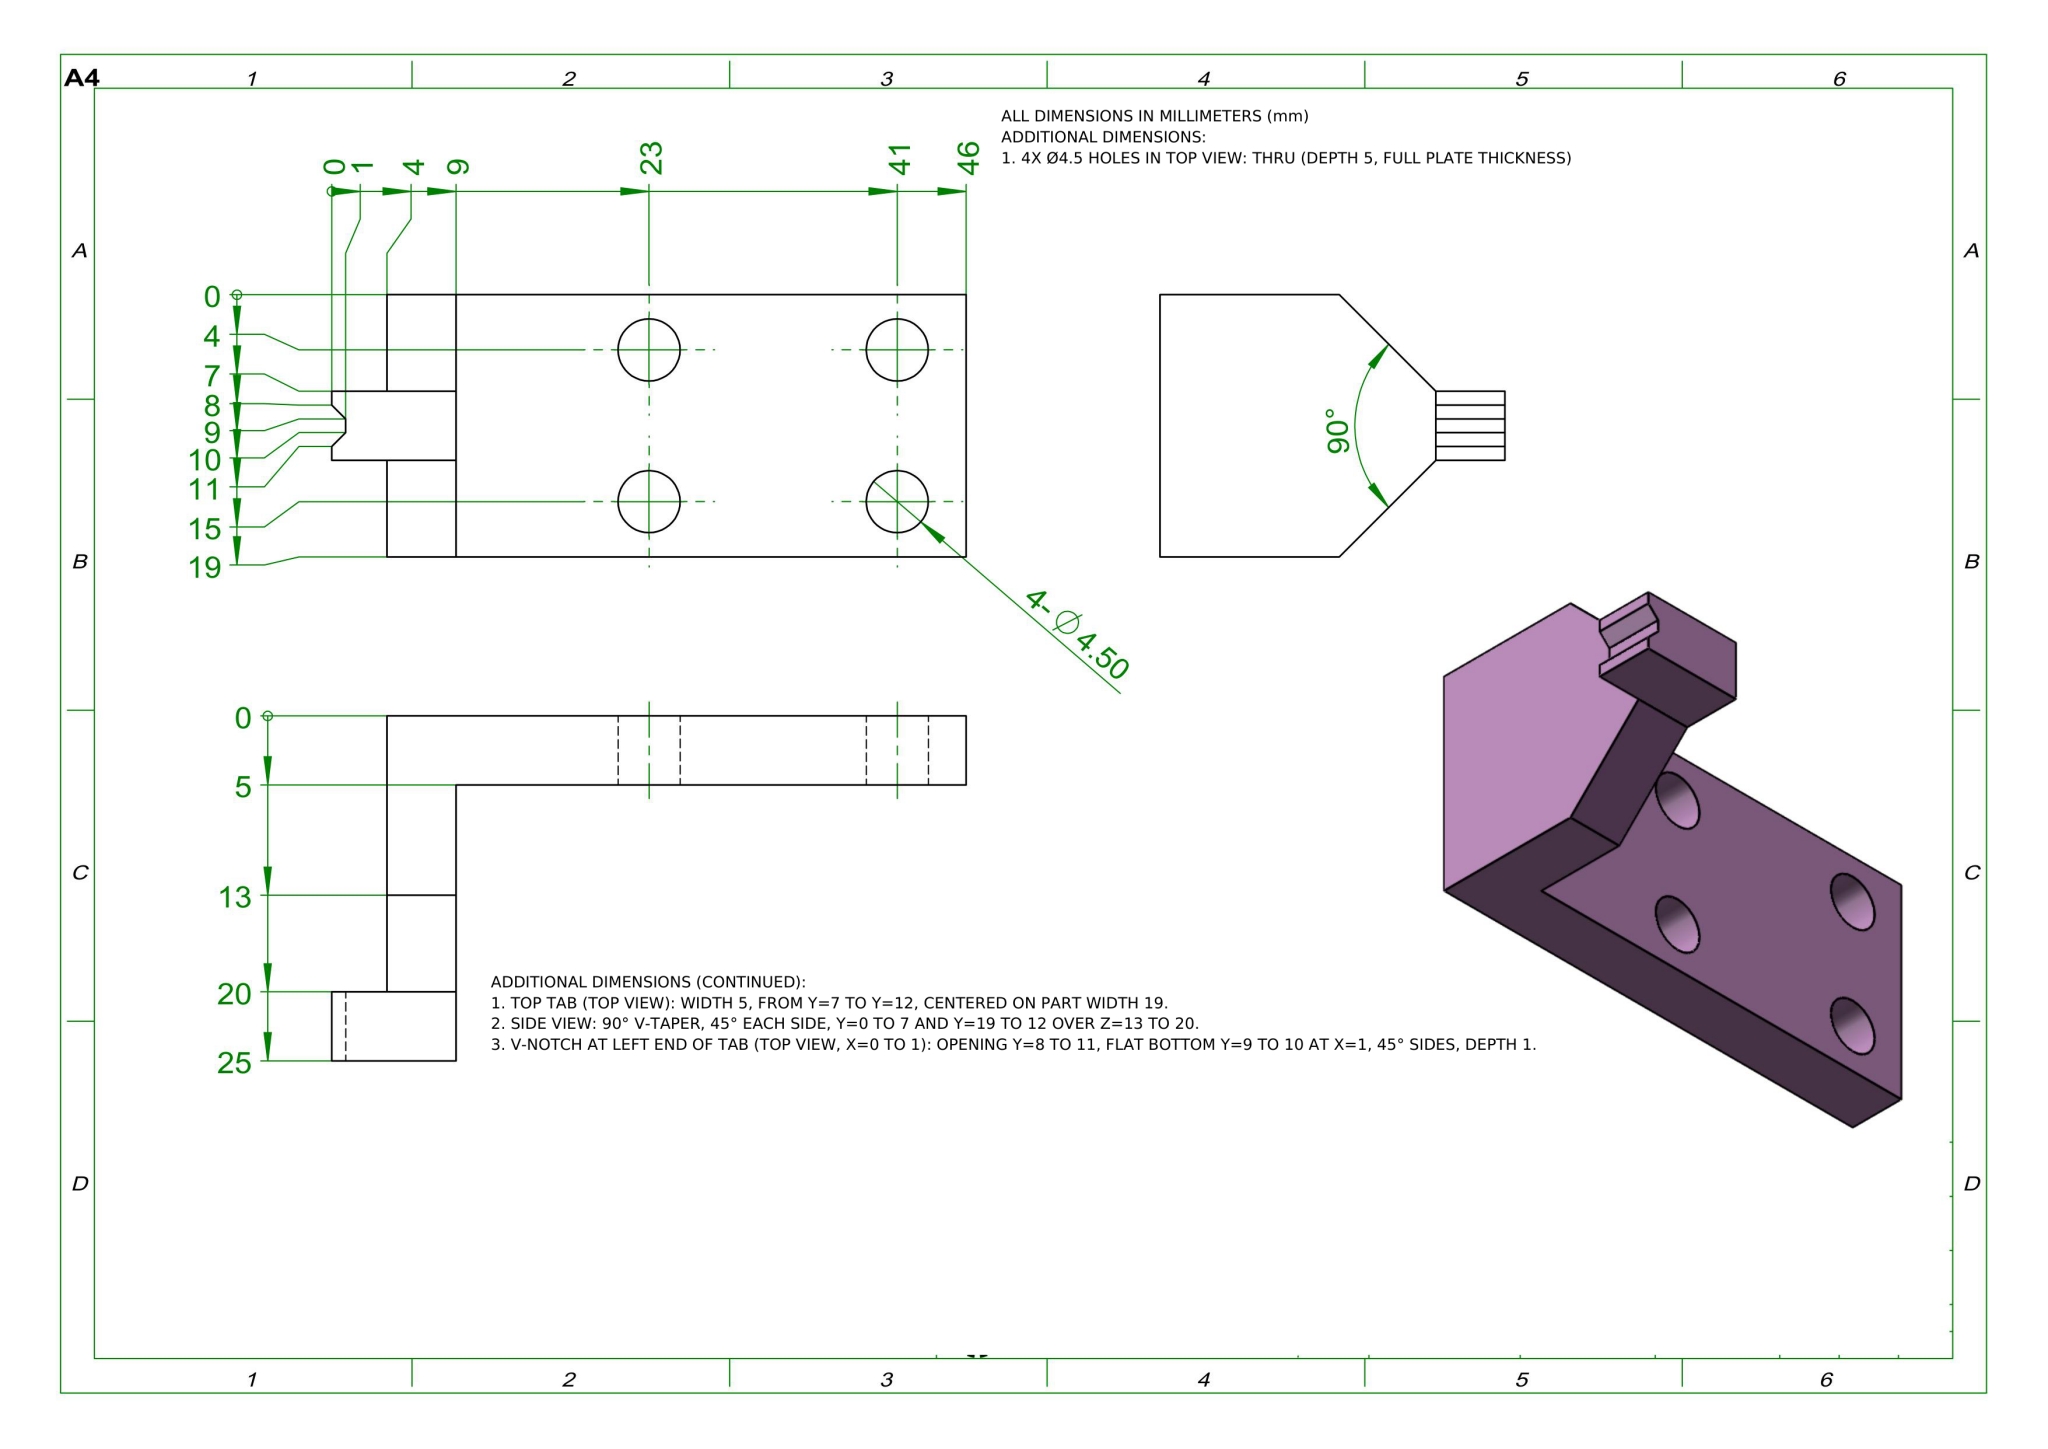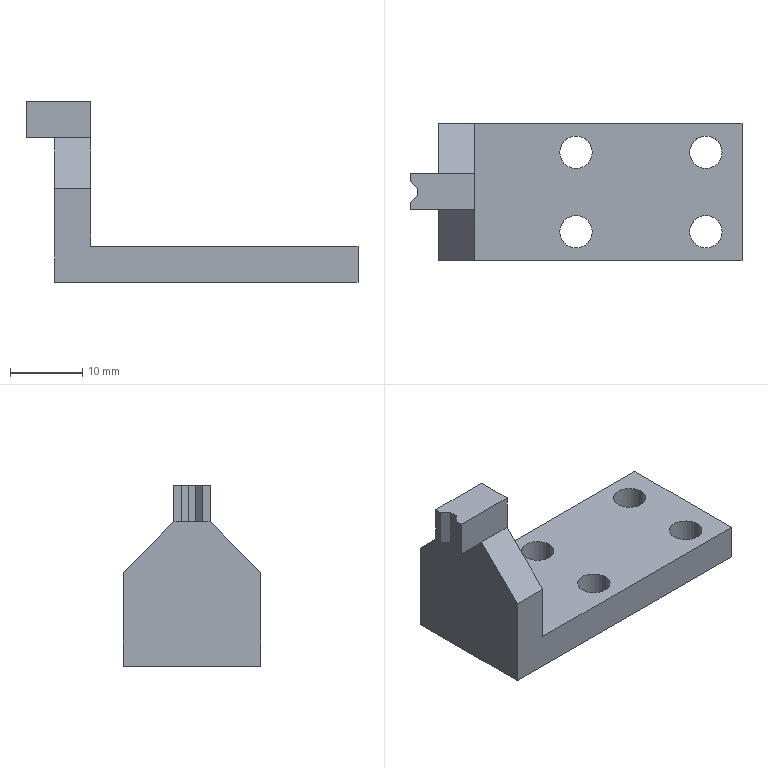Part | NX | mm | 1 solid | 26 faces | box 46 x 19 x 25 mm | volume 5067 mm3 | plane 18 | cylinder 8 | commonest cylinder face diameters 4.5 x8
STEP:
#1=COLOUR_RGB('',1.,0.7529,1.);
#2=FILL_AREA_STYLE_COLOUR('',#1);
#3=FILL_AREA_STYLE('',(#2));
#4=SURFACE_STYLE_FILL_AREA(#3);
#5=SURFACE_SIDE_STYLE('',(#4));
#6=SURFACE_STYLE_USAGE(.BOTH.,#5);
#7=PRESENTATION_STYLE_ASSIGNMENT((#6));
#8=CARTESIAN_POINT('',(-4.25,-5.5,0.));
#9=VERTEX_POINT('',#8);
#10=CARTESIAN_POINT('',(0.25,-5.5,0.));
#11=VERTEX_POINT('',#10);
#12=CARTESIAN_POINT('',(-2.,-5.5,0.));
#13=DIRECTION('',(0.,0.,1.));
#14=DIRECTION('',(-1.,0.,0.));
#15=AXIS2_PLACEMENT_3D('',#12,#13,#14);
#16=CIRCLE('',#15,2.25);
#17=EDGE_CURVE('',#9,#11,#16,.T.);
#18=ORIENTED_EDGE('',*,*,#17,.F.);
#19=CARTESIAN_POINT('',(-4.25,-5.5,5.));
#20=VERTEX_POINT('',#19);
#21=CARTESIAN_POINT('',(-4.25,-5.5,0.));
#22=DIRECTION('',(0.,0.,1.));
#23=VECTOR('',#22,1000.);
#24=LINE('',#21,#23);
#25=EDGE_CURVE('',#9,#20,#24,.T.);
#26=ORIENTED_EDGE('',*,*,#25,.T.);
#27=CARTESIAN_POINT('',(0.25,-5.5,5.));
#28=VERTEX_POINT('',#27);
#29=CARTESIAN_POINT('',(-2.,-5.5,5.));
#30=DIRECTION('',(0.,0.,1.));
#31=DIRECTION('',(-1.,0.,0.));
#32=AXIS2_PLACEMENT_3D('',#29,#30,#31);
#33=CIRCLE('',#32,2.25);
#34=EDGE_CURVE('',#20,#28,#33,.T.);
#35=ORIENTED_EDGE('',*,*,#34,.T.);
#36=CARTESIAN_POINT('',(0.25,-5.5,0.));
#37=DIRECTION('',(0.,0.,1.));
#38=VECTOR('',#37,1000.);
#39=LINE('',#36,#38);
#40=EDGE_CURVE('',#11,#28,#39,.T.);
#41=ORIENTED_EDGE('',*,*,#40,.F.);
#42=EDGE_LOOP('',(#18,#26,#35,#41));
#43=FACE_OUTER_BOUND('',#42,.T.);
#44=CARTESIAN_POINT('',(-2.,-5.5,0.));
#45=DIRECTION('',(0.,0.,1.));
#46=DIRECTION('',(1.,0.,0.));
#47=AXIS2_PLACEMENT_3D('',#44,#45,#46);
#48=CYLINDRICAL_SURFACE('',#47,2.25);
#49=ADVANCED_FACE('',(#43),#48,.F.);
#50=CARTESIAN_POINT('',(13.75,-5.5,0.));
#51=VERTEX_POINT('',#50);
#52=CARTESIAN_POINT('',(18.25,-5.5,0.));
#53=VERTEX_POINT('',#52);
#54=CARTESIAN_POINT('',(16.,-5.5,0.));
#55=DIRECTION('',(0.,0.,1.));
#56=DIRECTION('',(-1.,0.,0.));
#57=AXIS2_PLACEMENT_3D('',#54,#55,#56);
#58=CIRCLE('',#57,2.25);
#59=EDGE_CURVE('',#51,#53,#58,.T.);
#60=ORIENTED_EDGE('',*,*,#59,.F.);
#61=CARTESIAN_POINT('',(13.75,-5.5,5.));
#62=VERTEX_POINT('',#61);
#63=CARTESIAN_POINT('',(13.75,-5.5,0.));
#64=DIRECTION('',(0.,0.,1.));
#65=VECTOR('',#64,1000.);
#66=LINE('',#63,#65);
#67=EDGE_CURVE('',#51,#62,#66,.T.);
#68=ORIENTED_EDGE('',*,*,#67,.T.);
#69=CARTESIAN_POINT('',(18.25,-5.5,5.));
#70=VERTEX_POINT('',#69);
#71=CARTESIAN_POINT('',(16.,-5.5,5.));
#72=DIRECTION('',(0.,0.,1.));
#73=DIRECTION('',(-1.,0.,0.));
#74=AXIS2_PLACEMENT_3D('',#71,#72,#73);
#75=CIRCLE('',#74,2.25);
#76=EDGE_CURVE('',#62,#70,#75,.T.);
#77=ORIENTED_EDGE('',*,*,#76,.T.);
#78=CARTESIAN_POINT('',(18.25,-5.5,0.));
#79=DIRECTION('',(0.,0.,1.));
#80=VECTOR('',#79,1000.);
#81=LINE('',#78,#80);
#82=EDGE_CURVE('',#53,#70,#81,.T.);
#83=ORIENTED_EDGE('',*,*,#82,.F.);
#84=EDGE_LOOP('',(#60,#68,#77,#83));
#85=FACE_OUTER_BOUND('',#84,.T.);
#86=CARTESIAN_POINT('',(16.,-5.5,0.));
#87=DIRECTION('',(0.,0.,1.));
#88=DIRECTION('',(1.,0.,0.));
#89=AXIS2_PLACEMENT_3D('',#86,#87,#88);
#90=CYLINDRICAL_SURFACE('',#89,2.25);
#91=ADVANCED_FACE('',(#85),#90,.F.);
#92=CARTESIAN_POINT('',(13.75,5.5,0.));
#93=VERTEX_POINT('',#92);
#94=CARTESIAN_POINT('',(18.25,5.5,0.));
#95=VERTEX_POINT('',#94);
#96=CARTESIAN_POINT('',(16.,5.5,0.));
#97=DIRECTION('',(0.,0.,1.));
#98=DIRECTION('',(1.,0.,0.));
#99=AXIS2_PLACEMENT_3D('',#96,#97,#98);
#100=CIRCLE('',#99,2.25);
#101=EDGE_CURVE('',#93,#95,#100,.T.);
#102=ORIENTED_EDGE('',*,*,#101,.F.);
#103=CARTESIAN_POINT('',(13.75,5.5,5.));
#104=VERTEX_POINT('',#103);
#105=CARTESIAN_POINT('',(13.75,5.5,0.));
#106=DIRECTION('',(0.,0.,1.));
#107=VECTOR('',#106,1000.);
#108=LINE('',#105,#107);
#109=EDGE_CURVE('',#93,#104,#108,.T.);
#110=ORIENTED_EDGE('',*,*,#109,.T.);
#111=CARTESIAN_POINT('',(18.25,5.5,5.));
#112=VERTEX_POINT('',#111);
#113=CARTESIAN_POINT('',(16.,5.5,5.));
#114=DIRECTION('',(0.,0.,1.));
#115=DIRECTION('',(1.,0.,0.));
#116=AXIS2_PLACEMENT_3D('',#113,#114,#115);
#117=CIRCLE('',#116,2.25);
#118=EDGE_CURVE('',#104,#112,#117,.T.);
#119=ORIENTED_EDGE('',*,*,#118,.T.);
#120=CARTESIAN_POINT('',(18.25,5.5,0.));
#121=DIRECTION('',(0.,0.,1.));
#122=VECTOR('',#121,1000.);
#123=LINE('',#120,#122);
#124=EDGE_CURVE('',#95,#112,#123,.T.);
#125=ORIENTED_EDGE('',*,*,#124,.F.);
#126=EDGE_LOOP('',(#102,#110,#119,#125));
#127=FACE_OUTER_BOUND('',#126,.T.);
#128=CARTESIAN_POINT('',(16.,5.5,0.));
#129=DIRECTION('',(0.,0.,1.));
#130=DIRECTION('',(1.,0.,0.));
#131=AXIS2_PLACEMENT_3D('',#128,#129,#130);
#132=CYLINDRICAL_SURFACE('',#131,2.25);
#133=ADVANCED_FACE('',(#127),#132,.F.);
#134=CARTESIAN_POINT('',(-4.25,5.5,0.));
#135=VERTEX_POINT('',#134);
#136=CARTESIAN_POINT('',(0.25,5.5,0.));
#137=VERTEX_POINT('',#136);
#138=CARTESIAN_POINT('',(-2.,5.5,0.));
#139=DIRECTION('',(0.,0.,1.));
#140=DIRECTION('',(1.,0.,0.));
#141=AXIS2_PLACEMENT_3D('',#138,#139,#140);
#142=CIRCLE('',#141,2.25);
#143=EDGE_CURVE('',#135,#137,#142,.T.);
#144=ORIENTED_EDGE('',*,*,#143,.F.);
#145=CARTESIAN_POINT('',(-4.25,5.5,5.));
#146=VERTEX_POINT('',#145);
#147=CARTESIAN_POINT('',(-4.25,5.5,0.));
#148=DIRECTION('',(0.,0.,1.));
#149=VECTOR('',#148,1000.);
#150=LINE('',#147,#149);
#151=EDGE_CURVE('',#135,#146,#150,.T.);
#152=ORIENTED_EDGE('',*,*,#151,.T.);
#153=CARTESIAN_POINT('',(0.25,5.5,5.));
#154=VERTEX_POINT('',#153);
#155=CARTESIAN_POINT('',(-2.,5.5,5.));
#156=DIRECTION('',(0.,0.,1.));
#157=DIRECTION('',(1.,0.,0.));
#158=AXIS2_PLACEMENT_3D('',#155,#156,#157);
#159=CIRCLE('',#158,2.25);
#160=EDGE_CURVE('',#146,#154,#159,.T.);
#161=ORIENTED_EDGE('',*,*,#160,.T.);
#162=CARTESIAN_POINT('',(0.25,5.5,0.));
#163=DIRECTION('',(0.,0.,1.));
#164=VECTOR('',#163,1000.);
#165=LINE('',#162,#164);
#166=EDGE_CURVE('',#137,#154,#165,.T.);
#167=ORIENTED_EDGE('',*,*,#166,.F.);
#168=EDGE_LOOP('',(#144,#152,#161,#167));
#169=FACE_OUTER_BOUND('',#168,.T.);
#170=CARTESIAN_POINT('',(-2.,5.5,0.));
#171=DIRECTION('',(0.,0.,1.));
#172=DIRECTION('',(1.,0.,0.));
#173=AXIS2_PLACEMENT_3D('',#170,#171,#172);
#174=CYLINDRICAL_SURFACE('',#173,2.25);
#175=ADVANCED_FACE('',(#169),#174,.F.);
#176=CARTESIAN_POINT('',(-25.,-1.5,20.));
#177=VERTEX_POINT('',#176);
#178=CARTESIAN_POINT('',(-25.,-1.5,25.));
#179=VERTEX_POINT('',#178);
#180=CARTESIAN_POINT('',(-25.,-1.5,20.));
#181=DIRECTION('',(0.,0.,1.));
#182=VECTOR('',#181,1000.);
#183=LINE('',#180,#182);
#184=EDGE_CURVE('',#177,#179,#183,.T.);
#185=ORIENTED_EDGE('',*,*,#184,.F.);
#186=CARTESIAN_POINT('',(-25.,-2.5,20.));
#187=VERTEX_POINT('',#186);
#188=CARTESIAN_POINT('',(-25.,-2.5,20.));
#189=DIRECTION('',(0.,-1.,0.));
#190=VECTOR('',#189,1000.);
#191=LINE('',#188,#190);
#192=EDGE_CURVE('',#177,#187,#191,.T.);
#193=ORIENTED_EDGE('',*,*,#192,.T.);
#194=CARTESIAN_POINT('',(-25.,-2.5,25.));
#195=VERTEX_POINT('',#194);
#196=CARTESIAN_POINT('',(-25.,-2.5,25.));
#197=DIRECTION('',(0.,0.,1.));
#198=VECTOR('',#197,1000.);
#199=LINE('',#196,#198);
#200=EDGE_CURVE('',#187,#195,#199,.T.);
#201=ORIENTED_EDGE('',*,*,#200,.T.);
#202=CARTESIAN_POINT('',(-25.,-2.5,25.));
#203=DIRECTION('',(0.,1.,0.));
#204=VECTOR('',#203,1000.);
#205=LINE('',#202,#204);
#206=EDGE_CURVE('',#195,#179,#205,.T.);
#207=ORIENTED_EDGE('',*,*,#206,.T.);
#208=EDGE_LOOP('',(#185,#193,#201,#207));
#209=FACE_OUTER_BOUND('',#208,.T.);
#210=CARTESIAN_POINT('',(-25.,0.,0.));
#211=DIRECTION('',(-1.,0.,0.));
#212=DIRECTION('',(0.,0.,1.));
#213=AXIS2_PLACEMENT_3D('',#210,#211,#212);
#214=PLANE('',#213);
#215=ADVANCED_FACE('',(#209),#214,.T.);
#216=CARTESIAN_POINT('',(-21.,-9.5,13.));
#217=VERTEX_POINT('',#216);
#218=CARTESIAN_POINT('',(-21.,-9.5,0.));
#219=VERTEX_POINT('',#218);
#220=CARTESIAN_POINT('',(-21.,-9.5,5.));
#221=DIRECTION('',(0.,0.,-1.));
#222=VECTOR('',#221,1000.);
#223=LINE('',#220,#222);
#224=EDGE_CURVE('',#217,#219,#223,.T.);
#225=ORIENTED_EDGE('',*,*,#224,.F.);
#226=CARTESIAN_POINT('',(-21.,-2.5,20.));
#227=VERTEX_POINT('',#226);
#228=CARTESIAN_POINT('',(-21.,-9.5,13.));
#229=DIRECTION('',(0.,0.7071,0.7071));
#230=VECTOR('',#229,1000.);
#231=LINE('',#228,#230);
#232=EDGE_CURVE('',#217,#227,#231,.T.);
#233=ORIENTED_EDGE('',*,*,#232,.T.);
#234=CARTESIAN_POINT('',(-21.,2.5,20.));
#235=VERTEX_POINT('',#234);
#236=CARTESIAN_POINT('',(-21.,-2.5,20.));
#237=DIRECTION('',(0.,-1.,0.));
#238=VECTOR('',#237,1000.);
#239=LINE('',#236,#238);
#240=EDGE_CURVE('',#235,#227,#239,.T.);
#241=ORIENTED_EDGE('',*,*,#240,.F.);
#242=CARTESIAN_POINT('',(-21.,9.5,13.));
#243=VERTEX_POINT('',#242);
#244=CARTESIAN_POINT('',(-21.,2.5,20.));
#245=DIRECTION('',(0.,0.7071,-0.7071));
#246=VECTOR('',#245,1000.);
#247=LINE('',#244,#246);
#248=EDGE_CURVE('',#235,#243,#247,.T.);
#249=ORIENTED_EDGE('',*,*,#248,.T.);
#250=CARTESIAN_POINT('',(-21.,9.5,0.));
#251=VERTEX_POINT('',#250);
#252=CARTESIAN_POINT('',(-21.,9.5,5.));
#253=DIRECTION('',(0.,0.,-1.));
#254=VECTOR('',#253,1000.);
#255=LINE('',#252,#254);
#256=EDGE_CURVE('',#243,#251,#255,.T.);
#257=ORIENTED_EDGE('',*,*,#256,.T.);
#258=CARTESIAN_POINT('',(-21.,-9.5,0.));
#259=DIRECTION('',(0.,-1.,0.));
#260=VECTOR('',#259,1000.);
#261=LINE('',#258,#260);
#262=EDGE_CURVE('',#251,#219,#261,.T.);
#263=ORIENTED_EDGE('',*,*,#262,.T.);
#264=EDGE_LOOP('',(#225,#233,#241,#249,#257,#263));
#265=FACE_OUTER_BOUND('',#264,.T.);
#266=CARTESIAN_POINT('',(-21.,-9.5,5.));
#267=DIRECTION('',(1.,0.,0.));
#268=DIRECTION('',(0.,0.,-1.));
#269=AXIS2_PLACEMENT_3D('',#266,#267,#268);
#270=PLANE('',#269);
#271=ADVANCED_FACE('',(#265),#270,.F.);
#272=CARTESIAN_POINT('',(-2.,-5.5,5.));
#273=DIRECTION('',(0.,0.,1.));
#274=DIRECTION('',(-1.,0.,0.));
#275=AXIS2_PLACEMENT_3D('',#272,#273,#274);
#276=CIRCLE('',#275,2.25);
#277=EDGE_CURVE('',#28,#20,#276,.T.);
#278=ORIENTED_EDGE('',*,*,#277,.F.);
#279=ORIENTED_EDGE('',*,*,#34,.F.);
#280=EDGE_LOOP('',(#278,#279));
#281=FACE_BOUND('',#280,.T.);
#282=CARTESIAN_POINT('',(16.,-5.5,5.));
#283=DIRECTION('',(0.,0.,1.));
#284=DIRECTION('',(-1.,0.,0.));
#285=AXIS2_PLACEMENT_3D('',#282,#283,#284);
#286=CIRCLE('',#285,2.25);
#287=EDGE_CURVE('',#70,#62,#286,.T.);
#288=ORIENTED_EDGE('',*,*,#287,.F.);
#289=ORIENTED_EDGE('',*,*,#76,.F.);
#290=EDGE_LOOP('',(#288,#289));
#291=FACE_BOUND('',#290,.T.);
#292=CARTESIAN_POINT('',(16.,5.5,5.));
#293=DIRECTION('',(0.,0.,1.));
#294=DIRECTION('',(1.,0.,0.));
#295=AXIS2_PLACEMENT_3D('',#292,#293,#294);
#296=CIRCLE('',#295,2.25);
#297=EDGE_CURVE('',#112,#104,#296,.T.);
#298=ORIENTED_EDGE('',*,*,#297,.F.);
#299=ORIENTED_EDGE('',*,*,#118,.F.);
#300=EDGE_LOOP('',(#298,#299));
#301=FACE_BOUND('',#300,.T.);
#302=CARTESIAN_POINT('',(-2.,5.5,5.));
#303=DIRECTION('',(0.,0.,1.));
#304=DIRECTION('',(1.,0.,0.));
#305=AXIS2_PLACEMENT_3D('',#302,#303,#304);
#306=CIRCLE('',#305,2.25);
#307=EDGE_CURVE('',#154,#146,#306,.T.);
#308=ORIENTED_EDGE('',*,*,#307,.F.);
#309=ORIENTED_EDGE('',*,*,#160,.F.);
#310=EDGE_LOOP('',(#308,#309));
#311=FACE_BOUND('',#310,.T.);
#312=CARTESIAN_POINT('',(-16.,-9.5,5.));
#313=VERTEX_POINT('',#312);
#314=CARTESIAN_POINT('',(-16.,9.5,5.));
#315=VERTEX_POINT('',#314);
#316=CARTESIAN_POINT('',(-16.,9.5,5.));
#317=DIRECTION('',(-0.,1.,0.));
#318=VECTOR('',#317,1000.);
#319=LINE('',#316,#318);
#320=EDGE_CURVE('',#313,#315,#319,.T.);
#321=ORIENTED_EDGE('',*,*,#320,.F.);
#322=CARTESIAN_POINT('',(21.,-9.5,5.));
#323=VERTEX_POINT('',#322);
#324=CARTESIAN_POINT('',(-21.,-9.5,5.));
#325=DIRECTION('',(1.,0.,0.));
#326=VECTOR('',#325,1000.);
#327=LINE('',#324,#326);
#328=EDGE_CURVE('',#313,#323,#327,.T.);
#329=ORIENTED_EDGE('',*,*,#328,.T.);
#330=CARTESIAN_POINT('',(21.,9.5,5.));
#331=VERTEX_POINT('',#330);
#332=CARTESIAN_POINT('',(21.,-9.5,5.));
#333=DIRECTION('',(0.,1.,0.));
#334=VECTOR('',#333,1000.);
#335=LINE('',#332,#334);
#336=EDGE_CURVE('',#323,#331,#335,.T.);
#337=ORIENTED_EDGE('',*,*,#336,.T.);
#338=CARTESIAN_POINT('',(-21.,9.5,5.));
#339=DIRECTION('',(-1.,0.,0.));
#340=VECTOR('',#339,1000.);
#341=LINE('',#338,#340);
#342=EDGE_CURVE('',#331,#315,#341,.T.);
#343=ORIENTED_EDGE('',*,*,#342,.T.);
#344=EDGE_LOOP('',(#321,#329,#337,#343));
#345=FACE_OUTER_BOUND('',#344,.T.);
#346=CARTESIAN_POINT('',(0.,0.,5.));
#347=DIRECTION('',(0.,0.,-1.));
#348=DIRECTION('',(-1.,0.,0.));
#349=AXIS2_PLACEMENT_3D('',#346,#347,#348);
#350=PLANE('',#349);
#351=ADVANCED_FACE('',(#281,#291,#301,#311,#345),#350,.F.);
#352=CARTESIAN_POINT('',(21.,-9.5,0.));
#353=VERTEX_POINT('',#352);
#354=CARTESIAN_POINT('',(21.,9.5,0.));
#355=VERTEX_POINT('',#354);
#356=CARTESIAN_POINT('',(21.,-9.5,0.));
#357=DIRECTION('',(0.,1.,0.));
#358=VECTOR('',#357,1000.);
#359=LINE('',#356,#358);
#360=EDGE_CURVE('',#353,#355,#359,.T.);
#361=ORIENTED_EDGE('',*,*,#360,.T.);
#362=CARTESIAN_POINT('',(21.,9.5,5.));
#363=DIRECTION('',(0.,0.,-1.));
#364=VECTOR('',#363,1000.);
#365=LINE('',#362,#364);
#366=EDGE_CURVE('',#331,#355,#365,.T.);
#367=ORIENTED_EDGE('',*,*,#366,.F.);
#368=ORIENTED_EDGE('',*,*,#336,.F.);
#369=CARTESIAN_POINT('',(21.,-9.5,5.));
#370=DIRECTION('',(0.,0.,-1.));
#371=VECTOR('',#370,1000.);
#372=LINE('',#369,#371);
#373=EDGE_CURVE('',#323,#353,#372,.T.);
#374=ORIENTED_EDGE('',*,*,#373,.T.);
#375=EDGE_LOOP('',(#361,#367,#368,#374));
#376=FACE_OUTER_BOUND('',#375,.T.);
#377=CARTESIAN_POINT('',(21.,-9.5,5.));
#378=DIRECTION('',(-1.,0.,0.));
#379=DIRECTION('',(0.,0.,1.));
#380=AXIS2_PLACEMENT_3D('',#377,#378,#379);
#381=PLANE('',#380);
#382=ADVANCED_FACE('',(#376),#381,.F.);
#383=ORIENTED_EDGE('',*,*,#256,.F.);
#384=CARTESIAN_POINT('',(-16.,9.5,13.));
#385=VERTEX_POINT('',#384);
#386=CARTESIAN_POINT('',(-21.,9.5,13.));
#387=DIRECTION('',(1.,0.,0.));
#388=VECTOR('',#387,1000.);
#389=LINE('',#386,#388);
#390=EDGE_CURVE('',#243,#385,#389,.T.);
#391=ORIENTED_EDGE('',*,*,#390,.T.);
#392=CARTESIAN_POINT('',(-16.,9.5,25.));
#393=DIRECTION('',(0.,0.,-1.));
#394=VECTOR('',#393,1000.);
#395=LINE('',#392,#394);
#396=EDGE_CURVE('',#385,#315,#395,.T.);
#397=ORIENTED_EDGE('',*,*,#396,.T.);
#398=ORIENTED_EDGE('',*,*,#342,.F.);
#399=ORIENTED_EDGE('',*,*,#366,.T.);
#400=CARTESIAN_POINT('',(-21.,9.5,0.));
#401=DIRECTION('',(-1.,0.,0.));
#402=VECTOR('',#401,1000.);
#403=LINE('',#400,#402);
#404=EDGE_CURVE('',#355,#251,#403,.T.);
#405=ORIENTED_EDGE('',*,*,#404,.T.);
#406=EDGE_LOOP('',(#383,#391,#397,#398,#399,#405));
#407=FACE_OUTER_BOUND('',#406,.T.);
#408=CARTESIAN_POINT('',(-21.,9.5,5.));
#409=DIRECTION('',(0.,-1.,0.));
#410=DIRECTION('',(0.,0.,-1.));
#411=AXIS2_PLACEMENT_3D('',#408,#409,#410);
#412=PLANE('',#411);
#413=ADVANCED_FACE('',(#407),#412,.F.);
#414=CARTESIAN_POINT('',(-16.,-9.5,13.));
#415=VERTEX_POINT('',#414);
#416=CARTESIAN_POINT('',(-16.,-9.5,25.));
#417=DIRECTION('',(0.,0.,-1.));
#418=VECTOR('',#417,1000.);
#419=LINE('',#416,#418);
#420=EDGE_CURVE('',#415,#313,#419,.T.);
#421=ORIENTED_EDGE('',*,*,#420,.F.);
#422=CARTESIAN_POINT('',(-21.,-9.5,13.));
#423=DIRECTION('',(-1.,0.,0.));
#424=VECTOR('',#423,1000.);
#425=LINE('',#422,#424);
#426=EDGE_CURVE('',#415,#217,#425,.T.);
#427=ORIENTED_EDGE('',*,*,#426,.T.);
#428=ORIENTED_EDGE('',*,*,#224,.T.);
#429=CARTESIAN_POINT('',(-21.,-9.5,0.));
#430=DIRECTION('',(1.,0.,0.));
#431=VECTOR('',#430,1000.);
#432=LINE('',#429,#431);
#433=EDGE_CURVE('',#219,#353,#432,.T.);
#434=ORIENTED_EDGE('',*,*,#433,.T.);
#435=ORIENTED_EDGE('',*,*,#373,.F.);
#436=ORIENTED_EDGE('',*,*,#328,.F.);
#437=EDGE_LOOP('',(#421,#427,#428,#434,#435,#436));
#438=FACE_OUTER_BOUND('',#437,.T.);
#439=CARTESIAN_POINT('',(-21.,-9.5,5.));
#440=DIRECTION('',(0.,1.,0.));
#441=DIRECTION('',(0.,0.,1.));
#442=AXIS2_PLACEMENT_3D('',#439,#440,#441);
#443=PLANE('',#442);
#444=ADVANCED_FACE('',(#438),#443,.F.);
#445=CARTESIAN_POINT('',(-2.,-5.5,0.));
#446=DIRECTION('',(0.,0.,1.));
#447=DIRECTION('',(-1.,0.,0.));
#448=AXIS2_PLACEMENT_3D('',#445,#446,#447);
#449=CIRCLE('',#448,2.25);
#450=EDGE_CURVE('',#11,#9,#449,.T.);
#451=ORIENTED_EDGE('',*,*,#450,.T.);
#452=ORIENTED_EDGE('',*,*,#17,.T.);
#453=EDGE_LOOP('',(#451,#452));
#454=FACE_BOUND('',#453,.T.);
#455=CARTESIAN_POINT('',(16.,-5.5,0.));
#456=DIRECTION('',(0.,0.,1.));
#457=DIRECTION('',(-1.,0.,0.));
#458=AXIS2_PLACEMENT_3D('',#455,#456,#457);
#459=CIRCLE('',#458,2.25);
#460=EDGE_CURVE('',#53,#51,#459,.T.);
#461=ORIENTED_EDGE('',*,*,#460,.T.);
#462=ORIENTED_EDGE('',*,*,#59,.T.);
#463=EDGE_LOOP('',(#461,#462));
#464=FACE_BOUND('',#463,.T.);
#465=CARTESIAN_POINT('',(16.,5.5,0.));
#466=DIRECTION('',(0.,0.,1.));
#467=DIRECTION('',(1.,0.,0.));
#468=AXIS2_PLACEMENT_3D('',#465,#466,#467);
#469=CIRCLE('',#468,2.25);
#470=EDGE_CURVE('',#95,#93,#469,.T.);
#471=ORIENTED_EDGE('',*,*,#470,.T.);
#472=ORIENTED_EDGE('',*,*,#101,.T.);
#473=EDGE_LOOP('',(#471,#472));
#474=FACE_BOUND('',#473,.T.);
#475=CARTESIAN_POINT('',(-2.,5.5,0.));
#476=DIRECTION('',(0.,0.,1.));
#477=DIRECTION('',(1.,0.,0.));
#478=AXIS2_PLACEMENT_3D('',#475,#476,#477);
#479=CIRCLE('',#478,2.25);
#480=EDGE_CURVE('',#137,#135,#479,.T.);
#481=ORIENTED_EDGE('',*,*,#480,.T.);
#482=ORIENTED_EDGE('',*,*,#143,.T.);
#483=EDGE_LOOP('',(#481,#482));
#484=FACE_BOUND('',#483,.T.);
#485=ORIENTED_EDGE('',*,*,#360,.F.);
#486=ORIENTED_EDGE('',*,*,#433,.F.);
#487=ORIENTED_EDGE('',*,*,#262,.F.);
#488=ORIENTED_EDGE('',*,*,#404,.F.);
#489=EDGE_LOOP('',(#485,#486,#487,#488));
#490=FACE_OUTER_BOUND('',#489,.T.);
#491=CARTESIAN_POINT('',(0.,0.,0.));
#492=DIRECTION('',(0.,0.,-1.));
#493=DIRECTION('',(-1.,0.,0.));
#494=AXIS2_PLACEMENT_3D('',#491,#492,#493);
#495=PLANE('',#494);
#496=ADVANCED_FACE('',(#454,#464,#474,#484,#490),#495,.T.);
#497=CARTESIAN_POINT('',(-16.,-2.5,25.));
#498=VERTEX_POINT('',#497);
#499=CARTESIAN_POINT('',(-16.,-2.5,20.));
#500=VERTEX_POINT('',#499);
#501=CARTESIAN_POINT('',(-16.,-2.5,25.));
#502=DIRECTION('',(0.,0.,-1.));
#503=VECTOR('',#502,1000.);
#504=LINE('',#501,#503);
#505=EDGE_CURVE('',#498,#500,#504,.T.);
#506=ORIENTED_EDGE('',*,*,#505,.T.);
#507=CARTESIAN_POINT('',(-16.,-9.5,13.));
#508=DIRECTION('',(0.,-0.7071,-0.7071));
#509=VECTOR('',#508,1000.);
#510=LINE('',#507,#509);
#511=EDGE_CURVE('',#500,#415,#510,.T.);
#512=ORIENTED_EDGE('',*,*,#511,.T.);
#513=ORIENTED_EDGE('',*,*,#420,.T.);
#514=ORIENTED_EDGE('',*,*,#320,.T.);
#515=ORIENTED_EDGE('',*,*,#396,.F.);
#516=CARTESIAN_POINT('',(-16.,2.5,20.));
#517=VERTEX_POINT('',#516);
#518=CARTESIAN_POINT('',(-16.,2.5,20.));
#519=DIRECTION('',(0.,-0.7071,0.7071));
#520=VECTOR('',#519,1000.);
#521=LINE('',#518,#520);
#522=EDGE_CURVE('',#385,#517,#521,.T.);
#523=ORIENTED_EDGE('',*,*,#522,.T.);
#524=CARTESIAN_POINT('',(-16.,2.5,25.));
#525=VERTEX_POINT('',#524);
#526=CARTESIAN_POINT('',(-16.,2.5,25.));
#527=DIRECTION('',(-0.,0.,1.));
#528=VECTOR('',#527,1000.);
#529=LINE('',#526,#528);
#530=EDGE_CURVE('',#517,#525,#529,.T.);
#531=ORIENTED_EDGE('',*,*,#530,.T.);
#532=CARTESIAN_POINT('',(-16.,9.5,25.));
#533=DIRECTION('',(-0.,1.,0.));
#534=VECTOR('',#533,1000.);
#535=LINE('',#532,#534);
#536=EDGE_CURVE('',#498,#525,#535,.T.);
#537=ORIENTED_EDGE('',*,*,#536,.F.);
#538=EDGE_LOOP('',(#506,#512,#513,#514,#515,#523,#531,#537));
#539=FACE_OUTER_BOUND('',#538,.T.);
#540=CARTESIAN_POINT('',(-16.,9.5,25.));
#541=DIRECTION('',(-1.,-0.,0.));
#542=DIRECTION('',(0.,-1.,0.));
#543=AXIS2_PLACEMENT_3D('',#540,#541,#542);
#544=PLANE('',#543);
#545=ADVANCED_FACE('',(#539),#544,.F.);
#546=CARTESIAN_POINT('',(-24.,-0.5,25.));
#547=VERTEX_POINT('',#546);
#548=CARTESIAN_POINT('',(-25.,-1.5,25.));
#549=DIRECTION('',(0.7071,0.7071,0.));
#550=VECTOR('',#549,1000.);
#551=LINE('',#548,#550);
#552=EDGE_CURVE('',#179,#547,#551,.T.);
#553=ORIENTED_EDGE('',*,*,#552,.F.);
#554=ORIENTED_EDGE('',*,*,#206,.F.);
#555=CARTESIAN_POINT('',(0.,-2.5,25.));
#556=DIRECTION('',(-1.,0.,0.));
#557=VECTOR('',#556,1000.);
#558=LINE('',#555,#557);
#559=EDGE_CURVE('',#498,#195,#558,.T.);
#560=ORIENTED_EDGE('',*,*,#559,.F.);
#561=ORIENTED_EDGE('',*,*,#536,.T.);
#562=CARTESIAN_POINT('',(-25.,2.5,25.));
#563=VERTEX_POINT('',#562);
#564=CARTESIAN_POINT('',(0.,2.5,25.));
#565=DIRECTION('',(1.,0.,0.));
#566=VECTOR('',#565,1000.);
#567=LINE('',#564,#566);
#568=EDGE_CURVE('',#563,#525,#567,.T.);
#569=ORIENTED_EDGE('',*,*,#568,.F.);
#570=CARTESIAN_POINT('',(-25.,1.5,25.));
#571=VERTEX_POINT('',#570);
#572=CARTESIAN_POINT('',(-25.,-2.5,25.));
#573=DIRECTION('',(0.,1.,0.));
#574=VECTOR('',#573,1000.);
#575=LINE('',#572,#574);
#576=EDGE_CURVE('',#571,#563,#575,.T.);
#577=ORIENTED_EDGE('',*,*,#576,.F.);
#578=CARTESIAN_POINT('',(-24.,0.5,25.));
#579=VERTEX_POINT('',#578);
#580=CARTESIAN_POINT('',(-25.,1.5,25.));
#581=DIRECTION('',(-0.7071,0.7071,0.));
#582=VECTOR('',#581,1000.);
#583=LINE('',#580,#582);
#584=EDGE_CURVE('',#579,#571,#583,.T.);
#585=ORIENTED_EDGE('',*,*,#584,.F.);
#586=CARTESIAN_POINT('',(-24.,0.5,25.));
#587=DIRECTION('',(0.,1.,0.));
#588=VECTOR('',#587,1000.);
#589=LINE('',#586,#588);
#590=EDGE_CURVE('',#547,#579,#589,.T.);
#591=ORIENTED_EDGE('',*,*,#590,.F.);
#592=EDGE_LOOP('',(#553,#554,#560,#561,#569,#577,#585,#591));
#593=FACE_OUTER_BOUND('',#592,.T.);
#594=CARTESIAN_POINT('',(0.,0.,25.));
#595=DIRECTION('',(0.,0.,1.));
#596=DIRECTION('',(1.,0.,0.));
#597=AXIS2_PLACEMENT_3D('',#594,#595,#596);
#598=PLANE('',#597);
#599=ADVANCED_FACE('',(#593),#598,.T.);
#600=CARTESIAN_POINT('',(-1.,2.5,20.));
#601=DIRECTION('',(-1.,0.,0.));
#602=VECTOR('',#601,1000.);
#603=LINE('',#600,#602);
#604=EDGE_CURVE('',#517,#235,#603,.T.);
#605=ORIENTED_EDGE('',*,*,#604,.T.);
#606=CARTESIAN_POINT('',(-25.,2.5,20.));
#607=VERTEX_POINT('',#606);
#608=CARTESIAN_POINT('',(-25.,2.5,20.));
#609=DIRECTION('',(1.,0.,0.));
#610=VECTOR('',#609,1000.);
#611=LINE('',#608,#610);
#612=EDGE_CURVE('',#607,#235,#611,.T.);
#613=ORIENTED_EDGE('',*,*,#612,.F.);
#614=CARTESIAN_POINT('',(-25.,2.5,25.));
#615=DIRECTION('',(0.,-0.,-1.));
#616=VECTOR('',#615,1000.);
#617=LINE('',#614,#616);
#618=EDGE_CURVE('',#563,#607,#617,.T.);
#619=ORIENTED_EDGE('',*,*,#618,.F.);
#620=ORIENTED_EDGE('',*,*,#568,.T.);
#621=ORIENTED_EDGE('',*,*,#530,.F.);
#622=EDGE_LOOP('',(#605,#613,#619,#620,#621));
#623=FACE_OUTER_BOUND('',#622,.T.);
#624=CARTESIAN_POINT('',(-1.,2.5,25.));
#625=DIRECTION('',(0.,-1.,0.));
#626=DIRECTION('',(0.,-0.,-1.));
#627=AXIS2_PLACEMENT_3D('',#624,#625,#626);
#628=PLANE('',#627);
#629=ADVANCED_FACE('',(#623),#628,.F.);
#630=ORIENTED_EDGE('',*,*,#559,.T.);
#631=ORIENTED_EDGE('',*,*,#200,.F.);
#632=CARTESIAN_POINT('',(-25.,-2.5,20.));
#633=DIRECTION('',(1.,0.,0.));
#634=VECTOR('',#633,1000.);
#635=LINE('',#632,#634);
#636=EDGE_CURVE('',#187,#227,#635,.T.);
#637=ORIENTED_EDGE('',*,*,#636,.T.);
#638=CARTESIAN_POINT('',(-1.,-2.5,20.));
#639=DIRECTION('',(-1.,0.,0.));
#640=VECTOR('',#639,1000.);
#641=LINE('',#638,#640);
#642=EDGE_CURVE('',#500,#227,#641,.T.);
#643=ORIENTED_EDGE('',*,*,#642,.F.);
#644=ORIENTED_EDGE('',*,*,#505,.F.);
#645=EDGE_LOOP('',(#630,#631,#637,#643,#644));
#646=FACE_OUTER_BOUND('',#645,.T.);
#647=CARTESIAN_POINT('',(-1.,-2.5,25.));
#648=DIRECTION('',(0.,1.,0.));
#649=DIRECTION('',(0.,0.,1.));
#650=AXIS2_PLACEMENT_3D('',#647,#648,#649);
#651=PLANE('',#650);
#652=ADVANCED_FACE('',(#646),#651,.F.);
#653=ORIENTED_EDGE('',*,*,#192,.F.);
#654=CARTESIAN_POINT('',(-24.,-0.5,20.));
#655=VERTEX_POINT('',#654);
#656=CARTESIAN_POINT('',(-25.,-1.5,20.));
#657=DIRECTION('',(0.7071,0.7071,0.));
#658=VECTOR('',#657,1000.);
#659=LINE('',#656,#658);
#660=EDGE_CURVE('',#177,#655,#659,.T.);
#661=ORIENTED_EDGE('',*,*,#660,.T.);
#662=CARTESIAN_POINT('',(-24.,0.5,20.));
#663=VERTEX_POINT('',#662);
#664=CARTESIAN_POINT('',(-24.,0.5,20.));
#665=DIRECTION('',(0.,1.,0.));
#666=VECTOR('',#665,1000.);
#667=LINE('',#664,#666);
#668=EDGE_CURVE('',#655,#663,#667,.T.);
#669=ORIENTED_EDGE('',*,*,#668,.T.);
#670=CARTESIAN_POINT('',(-25.,1.5,20.));
#671=VERTEX_POINT('',#670);
#672=CARTESIAN_POINT('',(-25.,1.5,20.));
#673=DIRECTION('',(-0.7071,0.7071,0.));
#674=VECTOR('',#673,1000.);
#675=LINE('',#672,#674);
#676=EDGE_CURVE('',#663,#671,#675,.T.);
#677=ORIENTED_EDGE('',*,*,#676,.T.);
#678=CARTESIAN_POINT('',(-25.,-2.5,20.));
#679=DIRECTION('',(0.,-1.,0.));
#680=VECTOR('',#679,1000.);
#681=LINE('',#678,#680);
#682=EDGE_CURVE('',#607,#671,#681,.T.);
#683=ORIENTED_EDGE('',*,*,#682,.F.);
#684=ORIENTED_EDGE('',*,*,#612,.T.);
#685=ORIENTED_EDGE('',*,*,#240,.T.);
#686=ORIENTED_EDGE('',*,*,#636,.F.);
#687=EDGE_LOOP('',(#653,#661,#669,#677,#683,#684,#685,#686));
#688=FACE_OUTER_BOUND('',#687,.T.);
#689=CARTESIAN_POINT('',(-25.,-2.5,20.));
#690=DIRECTION('',(0.,0.,1.));
#691=DIRECTION('',(1.,0.,0.));
#692=AXIS2_PLACEMENT_3D('',#689,#690,#691);
#693=PLANE('',#692);
#694=ADVANCED_FACE('',(#688),#693,.F.);
#695=CARTESIAN_POINT('',(-25.,1.5,20.));
#696=DIRECTION('',(0.,0.,1.));
#697=VECTOR('',#696,1000.);
#698=LINE('',#695,#697);
#699=EDGE_CURVE('',#671,#571,#698,.T.);
#700=ORIENTED_EDGE('',*,*,#699,.T.);
#701=ORIENTED_EDGE('',*,*,#576,.T.);
#702=ORIENTED_EDGE('',*,*,#618,.T.);
#703=ORIENTED_EDGE('',*,*,#682,.T.);
#704=EDGE_LOOP('',(#700,#701,#702,#703));
#705=FACE_OUTER_BOUND('',#704,.T.);
#706=CARTESIAN_POINT('',(-25.,0.,0.));
#707=DIRECTION('',(-1.,0.,0.));
#708=DIRECTION('',(0.,0.,1.));
#709=AXIS2_PLACEMENT_3D('',#706,#707,#708);
#710=PLANE('',#709);
#711=ADVANCED_FACE('',(#705),#710,.T.);
#712=ORIENTED_EDGE('',*,*,#552,.T.);
#713=CARTESIAN_POINT('',(-24.,-0.5,20.));
#714=DIRECTION('',(0.,0.,1.));
#715=VECTOR('',#714,1000.);
#716=LINE('',#713,#715);
#717=EDGE_CURVE('',#655,#547,#716,.T.);
#718=ORIENTED_EDGE('',*,*,#717,.F.);
#719=ORIENTED_EDGE('',*,*,#660,.F.);
#720=ORIENTED_EDGE('',*,*,#184,.T.);
#721=EDGE_LOOP('',(#712,#718,#719,#720));
#722=FACE_OUTER_BOUND('',#721,.T.);
#723=CARTESIAN_POINT('',(-25.,-1.5,20.));
#724=DIRECTION('',(0.7071,-0.7071,0.));
#725=DIRECTION('',(0.7071,0.7071,0.));
#726=AXIS2_PLACEMENT_3D('',#723,#724,#725);
#727=PLANE('',#726);
#728=ADVANCED_FACE('',(#722),#727,.F.);
#729=ORIENTED_EDGE('',*,*,#584,.T.);
#730=ORIENTED_EDGE('',*,*,#699,.F.);
#731=ORIENTED_EDGE('',*,*,#676,.F.);
#732=CARTESIAN_POINT('',(-24.,0.5,20.));
#733=DIRECTION('',(0.,0.,1.));
#734=VECTOR('',#733,1000.);
#735=LINE('',#732,#734);
#736=EDGE_CURVE('',#663,#579,#735,.T.);
#737=ORIENTED_EDGE('',*,*,#736,.T.);
#738=EDGE_LOOP('',(#729,#730,#731,#737));
#739=FACE_OUTER_BOUND('',#738,.T.);
#740=CARTESIAN_POINT('',(-25.,1.5,20.));
#741=DIRECTION('',(0.7071,0.7071,0.));
#742=DIRECTION('',(-0.7071,0.7071,0.));
#743=AXIS2_PLACEMENT_3D('',#740,#741,#742);
#744=PLANE('',#743);
#745=ADVANCED_FACE('',(#739),#744,.F.);
#746=ORIENTED_EDGE('',*,*,#590,.T.);
#747=ORIENTED_EDGE('',*,*,#736,.F.);
#748=ORIENTED_EDGE('',*,*,#668,.F.);
#749=ORIENTED_EDGE('',*,*,#717,.T.);
#750=EDGE_LOOP('',(#746,#747,#748,#749));
#751=FACE_OUTER_BOUND('',#750,.T.);
#752=CARTESIAN_POINT('',(-24.,0.5,20.));
#753=DIRECTION('',(1.,0.,0.));
#754=DIRECTION('',(0.,0.,-1.));
#755=AXIS2_PLACEMENT_3D('',#752,#753,#754);
#756=PLANE('',#755);
#757=ADVANCED_FACE('',(#751),#756,.F.);
#758=ORIENTED_EDGE('',*,*,#151,.F.);
#759=ORIENTED_EDGE('',*,*,#480,.F.);
#760=ORIENTED_EDGE('',*,*,#166,.T.);
#761=ORIENTED_EDGE('',*,*,#307,.T.);
#762=EDGE_LOOP('',(#758,#759,#760,#761));
#763=FACE_OUTER_BOUND('',#762,.T.);
#764=CARTESIAN_POINT('',(-2.,5.5,0.));
#765=DIRECTION('',(0.,0.,1.));
#766=DIRECTION('',(1.,0.,0.));
#767=AXIS2_PLACEMENT_3D('',#764,#765,#766);
#768=CYLINDRICAL_SURFACE('',#767,2.25);
#769=ADVANCED_FACE('',(#763),#768,.F.);
#770=ORIENTED_EDGE('',*,*,#109,.F.);
#771=ORIENTED_EDGE('',*,*,#470,.F.);
#772=ORIENTED_EDGE('',*,*,#124,.T.);
#773=ORIENTED_EDGE('',*,*,#297,.T.);
#774=EDGE_LOOP('',(#770,#771,#772,#773));
#775=FACE_OUTER_BOUND('',#774,.T.);
#776=CARTESIAN_POINT('',(16.,5.5,0.));
#777=DIRECTION('',(0.,0.,1.));
#778=DIRECTION('',(1.,0.,0.));
#779=AXIS2_PLACEMENT_3D('',#776,#777,#778);
#780=CYLINDRICAL_SURFACE('',#779,2.25);
#781=ADVANCED_FACE('',(#775),#780,.F.);
#782=ORIENTED_EDGE('',*,*,#67,.F.);
#783=ORIENTED_EDGE('',*,*,#460,.F.);
#784=ORIENTED_EDGE('',*,*,#82,.T.);
#785=ORIENTED_EDGE('',*,*,#287,.T.);
#786=EDGE_LOOP('',(#782,#783,#784,#785));
#787=FACE_OUTER_BOUND('',#786,.T.);
#788=CARTESIAN_POINT('',(16.,-5.5,0.));
#789=DIRECTION('',(0.,0.,1.));
#790=DIRECTION('',(1.,0.,0.));
#791=AXIS2_PLACEMENT_3D('',#788,#789,#790);
#792=CYLINDRICAL_SURFACE('',#791,2.25);
#793=ADVANCED_FACE('',(#787),#792,.F.);
#794=ORIENTED_EDGE('',*,*,#25,.F.);
#795=ORIENTED_EDGE('',*,*,#450,.F.);
#796=ORIENTED_EDGE('',*,*,#40,.T.);
#797=ORIENTED_EDGE('',*,*,#277,.T.);
#798=EDGE_LOOP('',(#794,#795,#796,#797));
#799=FACE_OUTER_BOUND('',#798,.T.);
#800=CARTESIAN_POINT('',(-2.,-5.5,0.));
#801=DIRECTION('',(0.,0.,1.));
#802=DIRECTION('',(1.,0.,0.));
#803=AXIS2_PLACEMENT_3D('',#800,#801,#802);
#804=CYLINDRICAL_SURFACE('',#803,2.25);
#805=ADVANCED_FACE('',(#799),#804,.F.);
#806=ORIENTED_EDGE('',*,*,#511,.F.);
#807=ORIENTED_EDGE('',*,*,#642,.T.);
#808=ORIENTED_EDGE('',*,*,#232,.F.);
#809=ORIENTED_EDGE('',*,*,#426,.F.);
#810=EDGE_LOOP('',(#806,#807,#808,#809));
#811=FACE_OUTER_BOUND('',#810,.T.);
#812=CARTESIAN_POINT('',(-21.,-9.5,13.));
#813=DIRECTION('',(0.,0.7071,-0.7071));
#814=DIRECTION('',(-1.,0.,0.));
#815=AXIS2_PLACEMENT_3D('',#812,#813,#814);
#816=PLANE('',#815);
#817=ADVANCED_FACE('',(#811),#816,.F.);
#818=ORIENTED_EDGE('',*,*,#522,.F.);
#819=ORIENTED_EDGE('',*,*,#390,.F.);
#820=ORIENTED_EDGE('',*,*,#248,.F.);
#821=ORIENTED_EDGE('',*,*,#604,.F.);
#822=EDGE_LOOP('',(#818,#819,#820,#821));
#823=FACE_OUTER_BOUND('',#822,.T.);
#824=CARTESIAN_POINT('',(-1.,2.5,20.));
#825=DIRECTION('',(0.,-0.7071,-0.7071));
#826=DIRECTION('',(-1.,0.,0.));
#827=AXIS2_PLACEMENT_3D('',#824,#825,#826);
#828=PLANE('',#827);
#829=ADVANCED_FACE('',(#823),#828,.F.);
#830=CLOSED_SHELL('',(#49,#91,#133,#175,#215,#271,#351,#382,#413,#444,#496,#545,#599,#629,#652,#694,#711,#728,#745,#757,#769,#781,#793,#805,#817,#829));
#831=MANIFOLD_SOLID_BREP('',#830);
#832=STYLED_ITEM('',(#7),#831);
#833=PRESENTATION_LAYER_ASSIGNMENT('','',(#832));
#834=(LENGTH_UNIT()NAMED_UNIT(*)SI_UNIT(.MILLI.,.METRE.));
#835=UNCERTAINTY_MEASURE_WITH_UNIT(LENGTH_MEASURE(0.00001),#834,'','');
#836=(NAMED_UNIT(*)PLANE_ANGLE_UNIT()SI_UNIT($,.RADIAN.));
#837=(NAMED_UNIT(*)SI_UNIT($,.STERADIAN.)SOLID_ANGLE_UNIT());
#838=(GEOMETRIC_REPRESENTATION_CONTEXT(3)GLOBAL_UNCERTAINTY_ASSIGNED_CONTEXT((#835))GLOBAL_UNIT_ASSIGNED_CONTEXT((#834,#836,#837))REPRESENTATION_CONTEXT('',''));
#839=MECHANICAL_DESIGN_GEOMETRIC_PRESENTATION_REPRESENTATION('',(#832),#838);
#840=COLOUR_RGB('',1.,0.7529,1.);
#841=FILL_AREA_STYLE_COLOUR('',#840);
#842=FILL_AREA_STYLE('',(#841));
#843=SURFACE_STYLE_FILL_AREA(#842);
#844=SURFACE_SIDE_STYLE('',(#843));
#845=SURFACE_STYLE_USAGE(.BOTH.,#844);
#846=PRESENTATION_STYLE_ASSIGNMENT((#845));
#847=CARTESIAN_POINT('',(0.,0.,0.));
#848=DIRECTION('',(0.,0.,1.));
#849=DIRECTION('',(1.,0.,0.));
#850=AXIS2_PLACEMENT_3D('',#847,#848,#849);
#851=(LENGTH_UNIT()NAMED_UNIT(*)SI_UNIT(.MILLI.,.METRE.));
#852=UNCERTAINTY_MEASURE_WITH_UNIT(LENGTH_MEASURE(0.00001),#851,'','');
#853=(NAMED_UNIT(*)PLANE_ANGLE_UNIT()SI_UNIT($,.RADIAN.));
#854=(NAMED_UNIT(*)SI_UNIT($,.STERADIAN.)SOLID_ANGLE_UNIT());
#855=(GEOMETRIC_REPRESENTATION_CONTEXT(3)GLOBAL_UNCERTAINTY_ASSIGNED_CONTEXT((#852))GLOBAL_UNIT_ASSIGNED_CONTEXT((#851,#853,#854))REPRESENTATION_CONTEXT('',''));
#856=ADVANCED_BREP_SHAPE_REPRESENTATION('',(#831,#850),#855);
#857=STYLED_ITEM('',(#846),#856);
#858=PRESENTATION_LAYER_ASSIGNMENT('','',(#857));
#859=(LENGTH_UNIT()NAMED_UNIT(*)SI_UNIT(.MILLI.,.METRE.));
#860=UNCERTAINTY_MEASURE_WITH_UNIT(LENGTH_MEASURE(0.00001),#859,'','');
#861=(NAMED_UNIT(*)PLANE_ANGLE_UNIT()SI_UNIT($,.RADIAN.));
#862=(NAMED_UNIT(*)SI_UNIT($,.STERADIAN.)SOLID_ANGLE_UNIT());
#863=(GEOMETRIC_REPRESENTATION_CONTEXT(3)GLOBAL_UNCERTAINTY_ASSIGNED_CONTEXT((#860))GLOBAL_UNIT_ASSIGNED_CONTEXT((#859,#861,#862))REPRESENTATION_CONTEXT('',''));
#864=MECHANICAL_DESIGN_GEOMETRIC_PRESENTATION_REPRESENTATION('',(#857),#863);